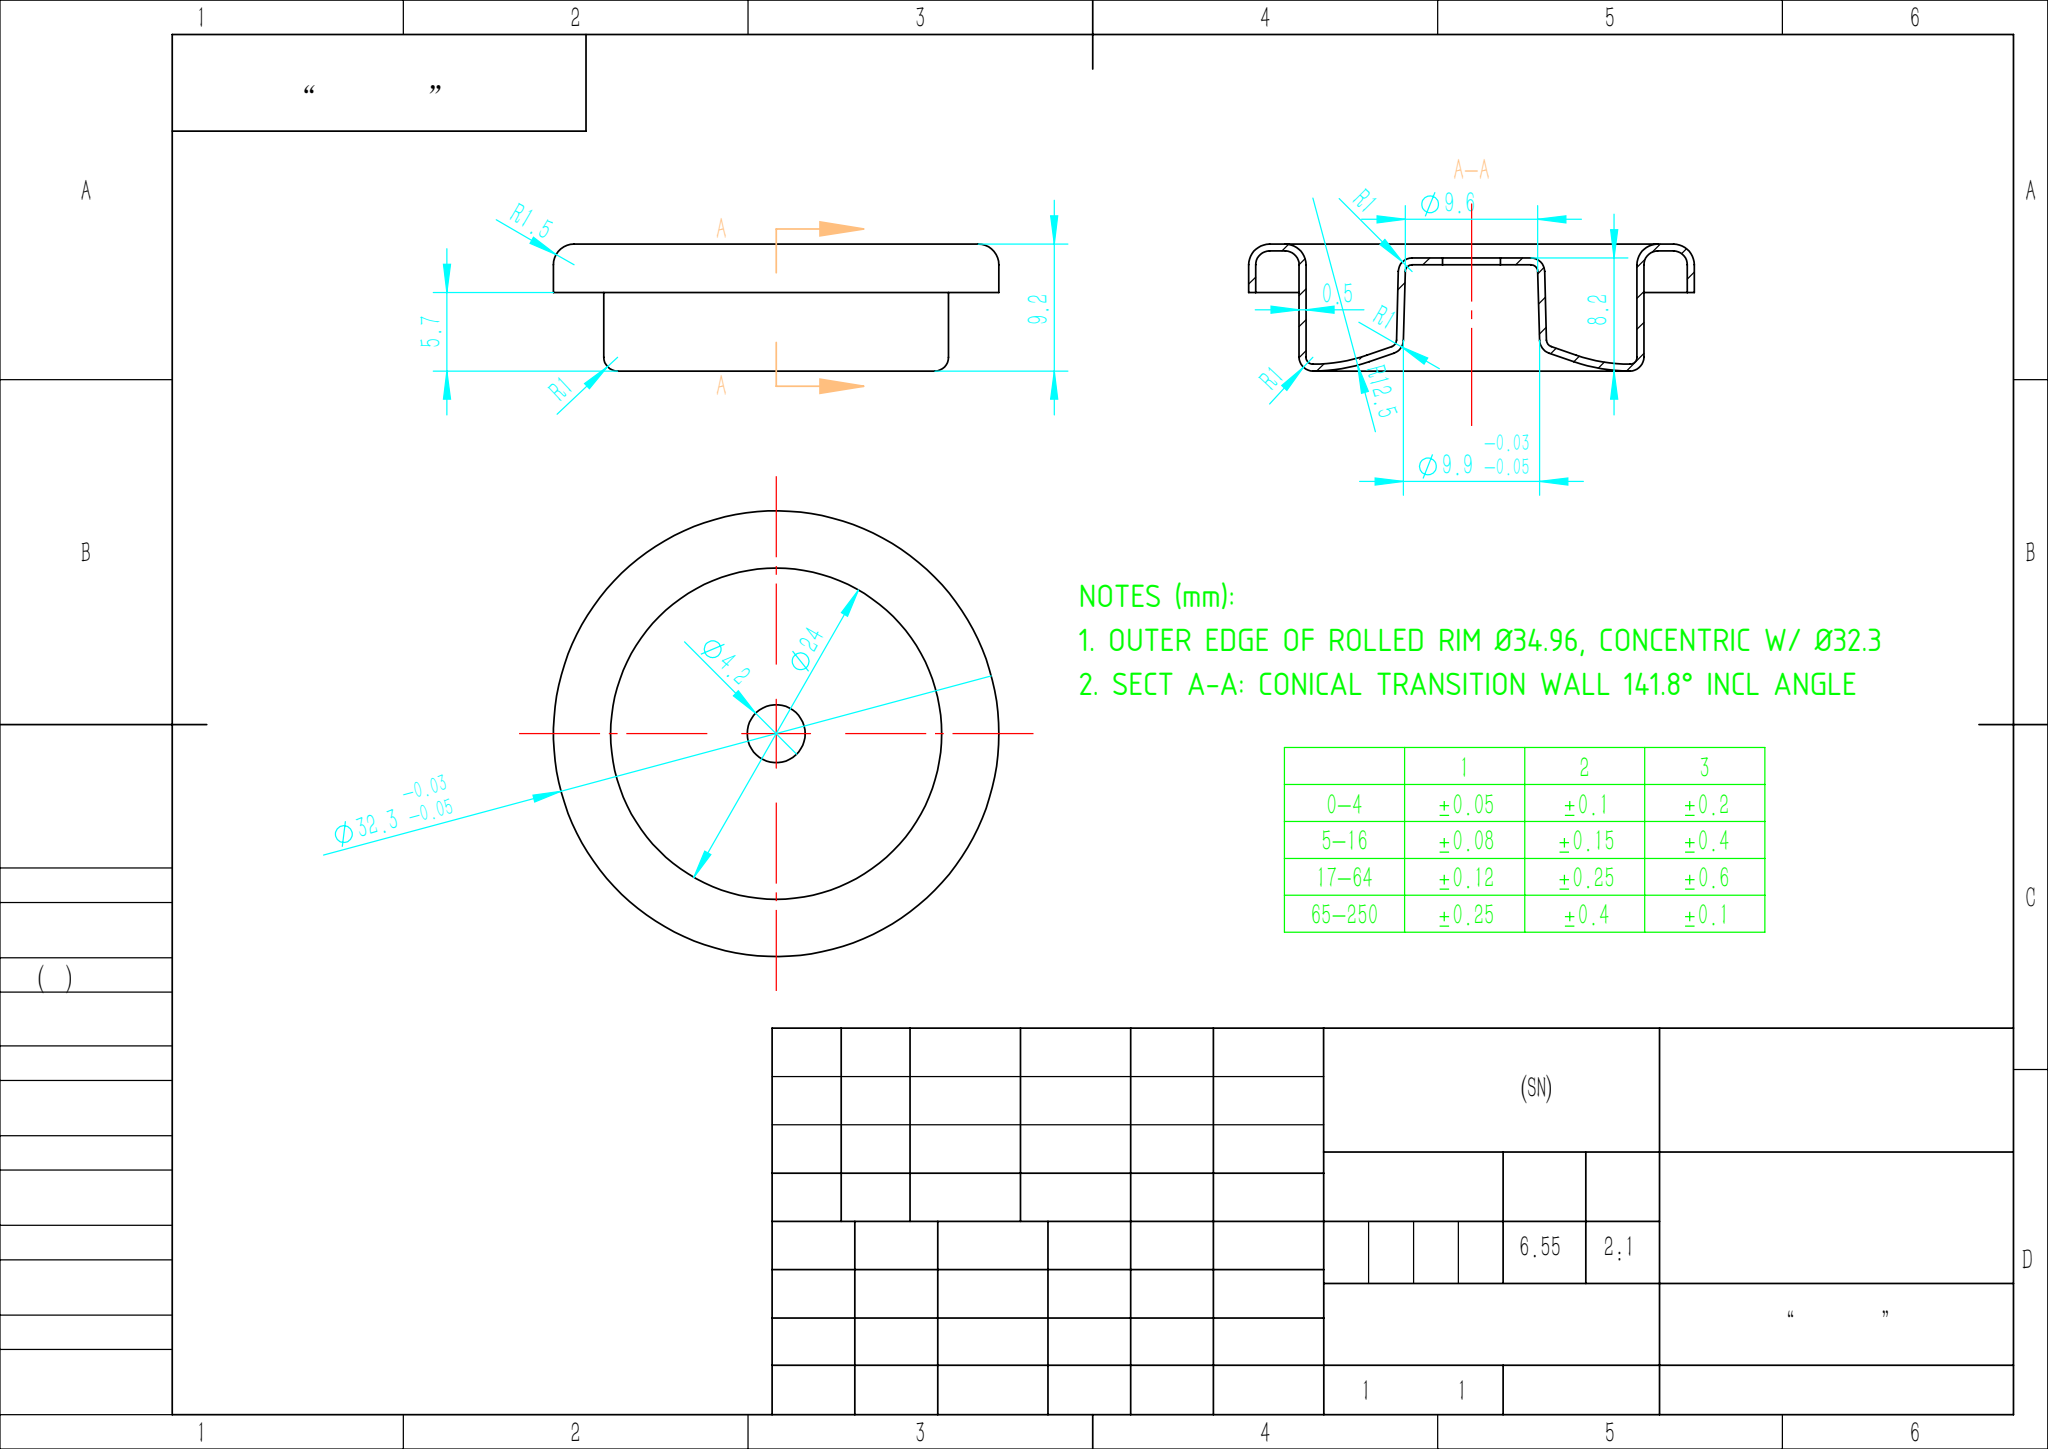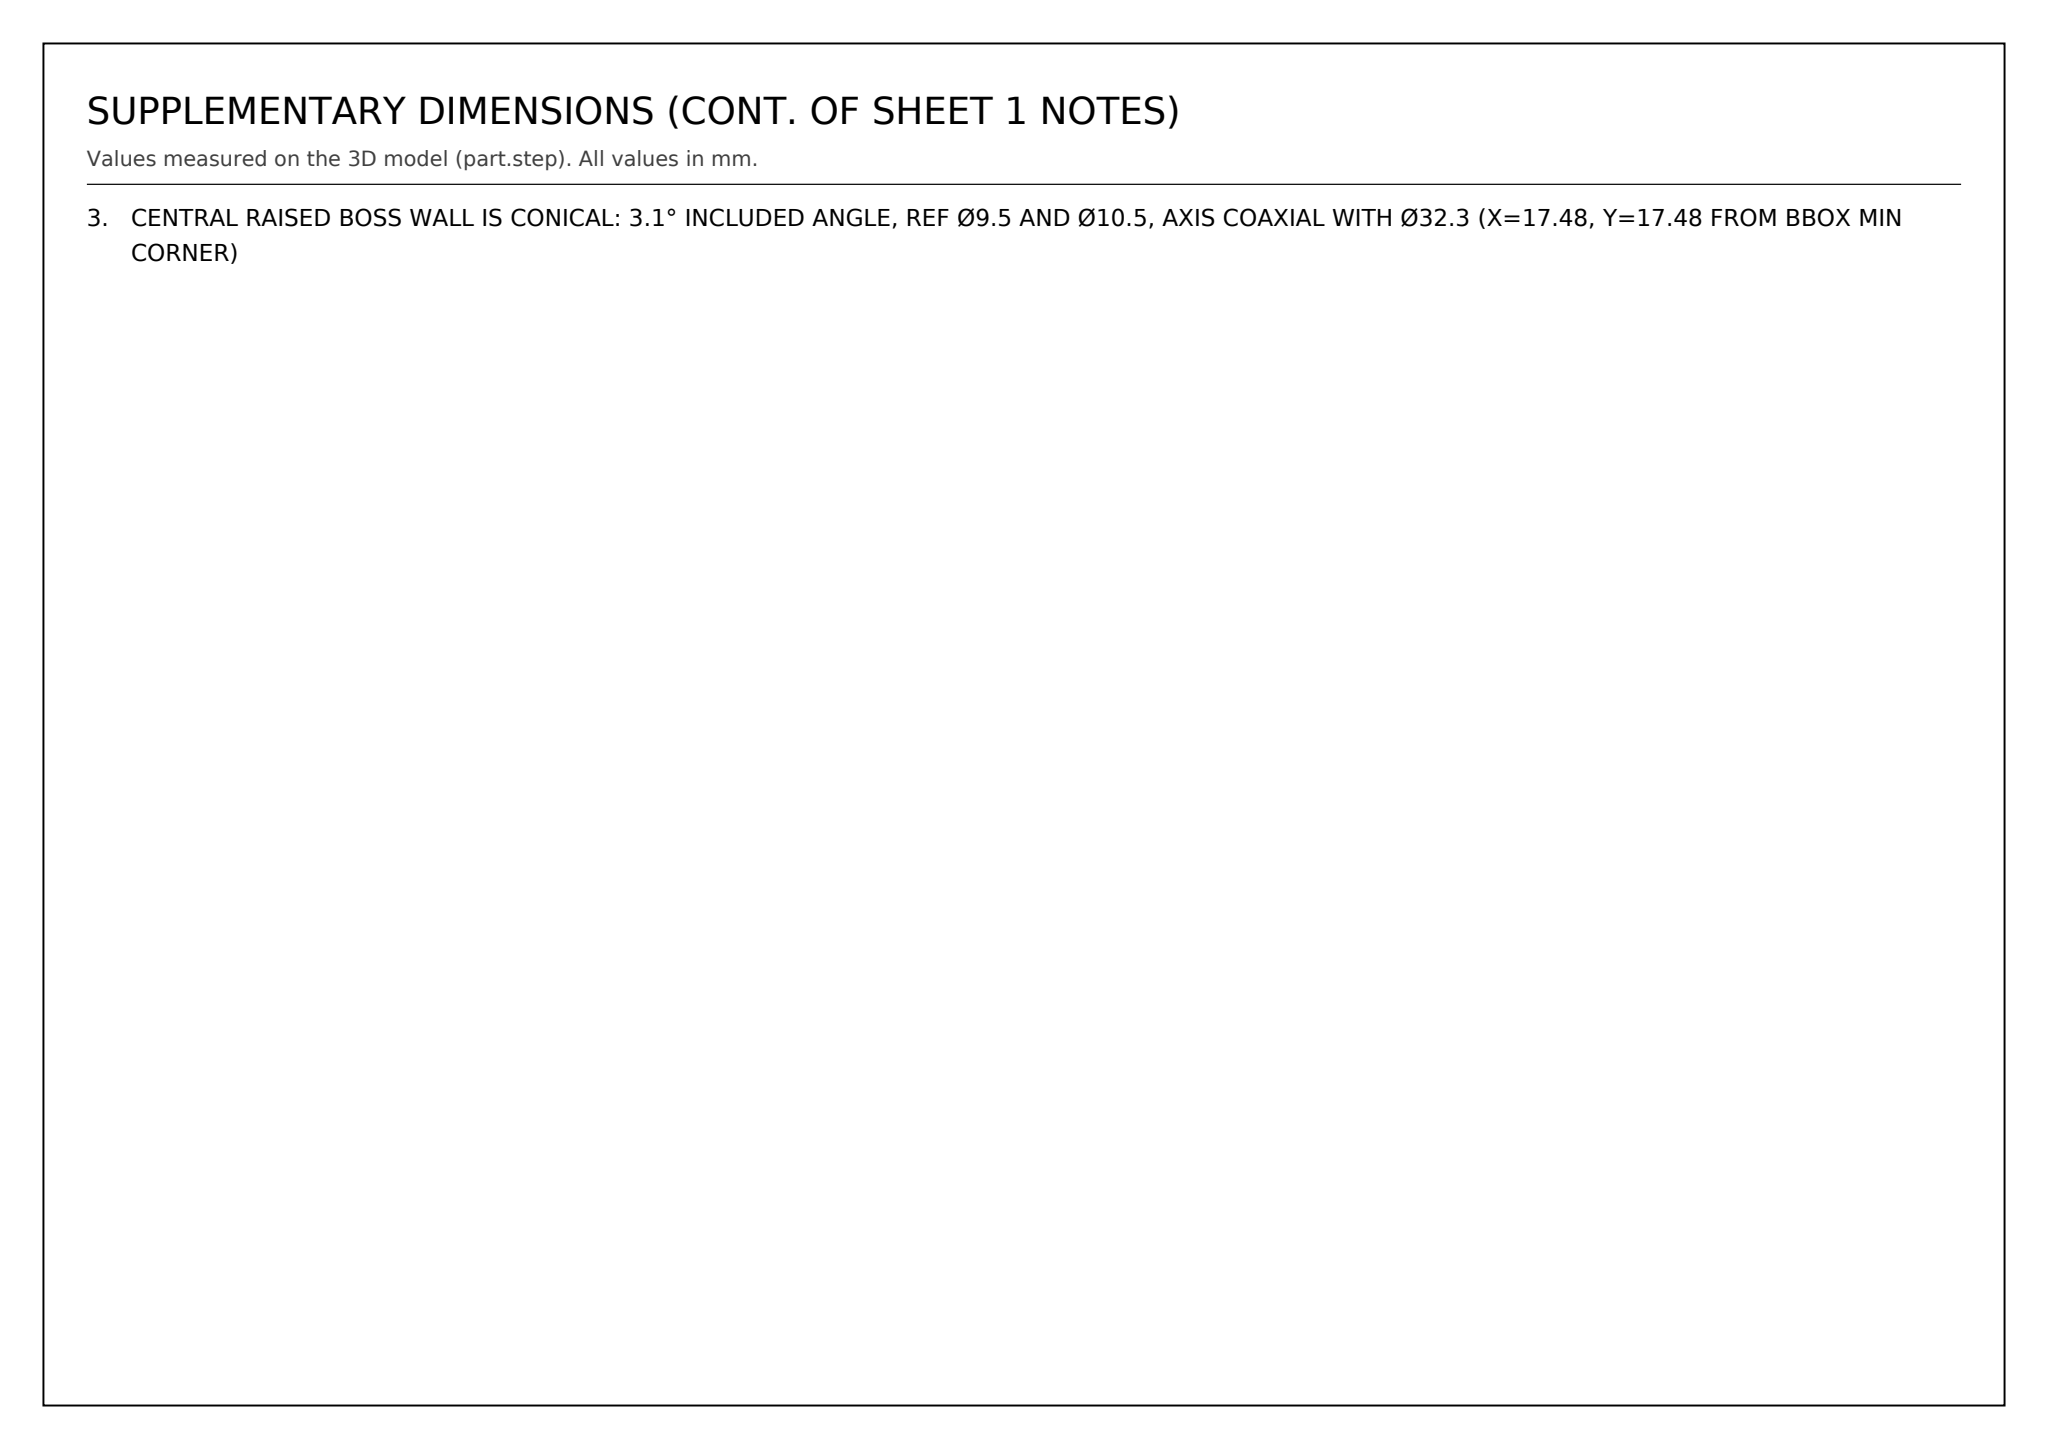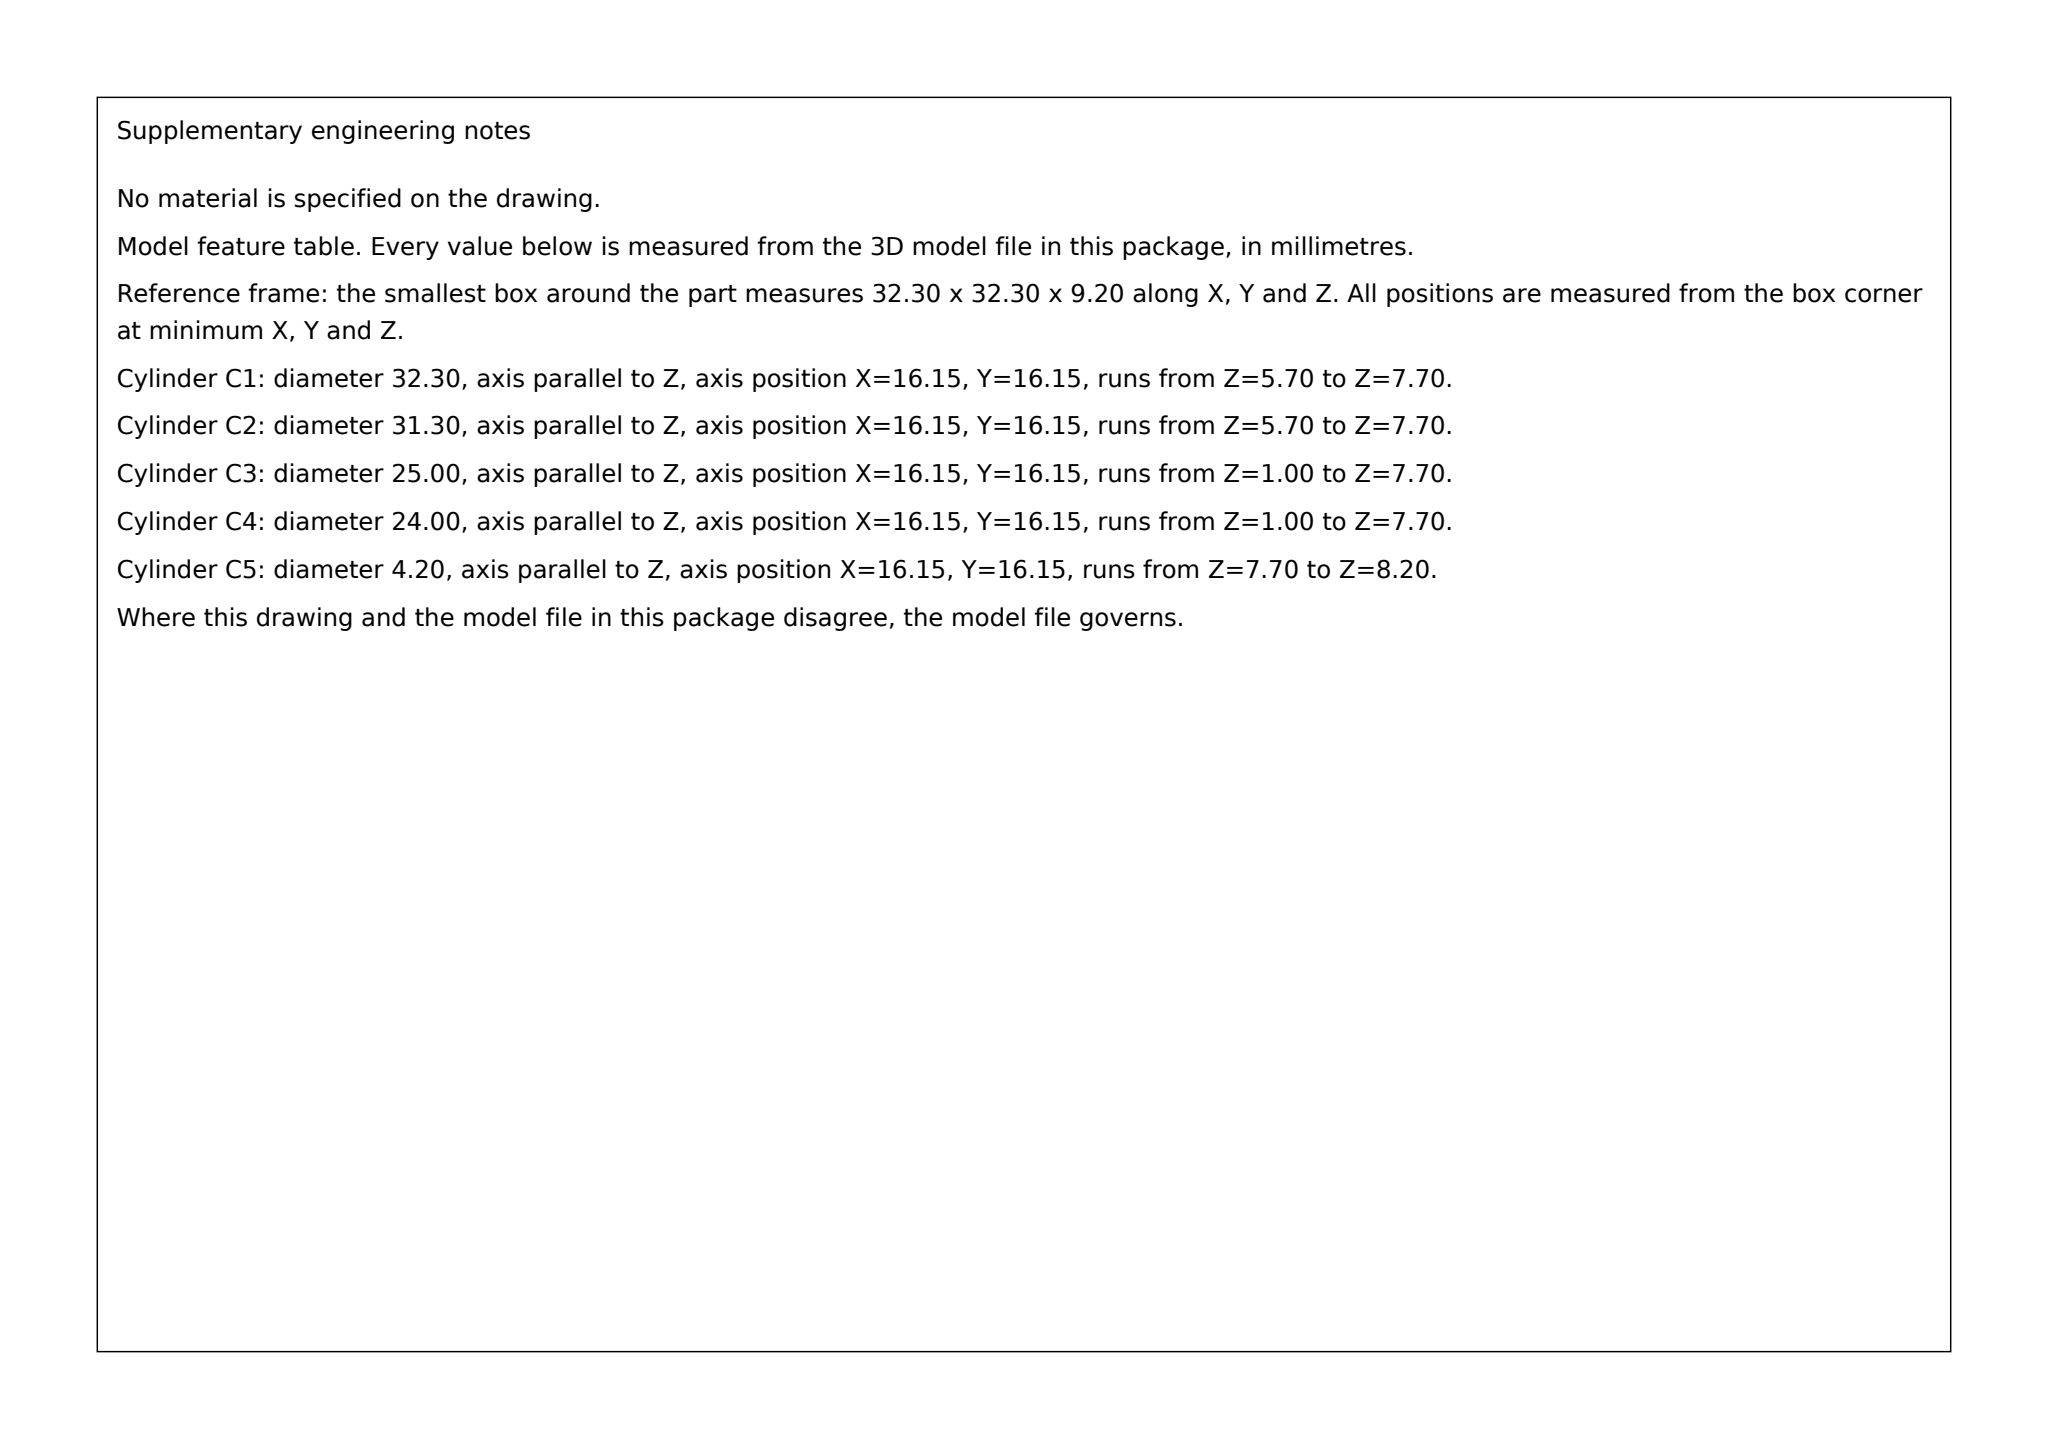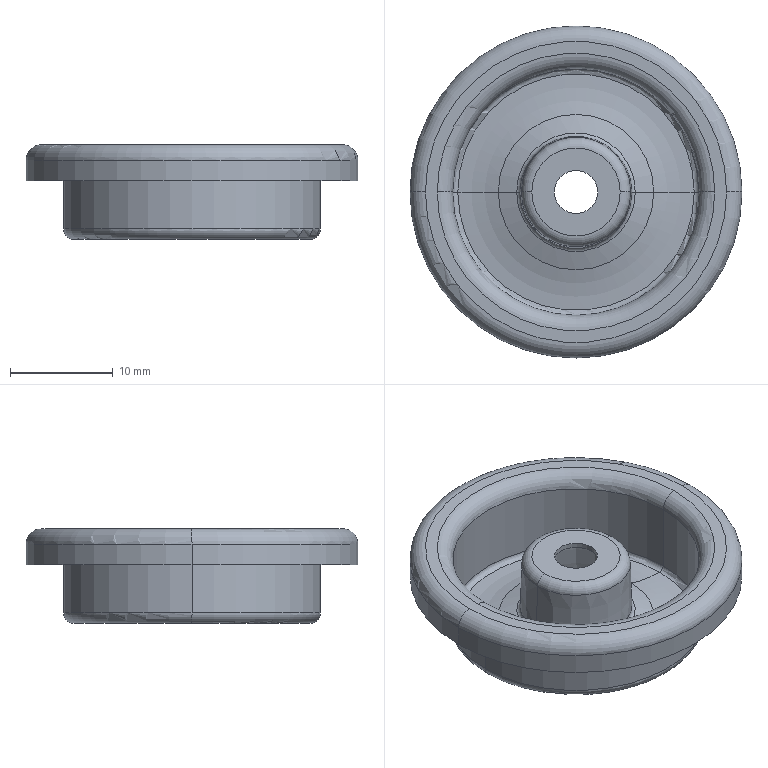Part | SolidWorks | mm | 1 solid | 47 faces | box 32.3 x 32.3 x 9.2 mm | volume 923 mm3 | torus 24 | cylinder 10 | cone 8 | plane 5 | commonest cylinder face diameters 4.2 x2 31.3 x2 32.3 x2 24 x2 25 x2
Drawing notes:
OUTER EDGE OF ROLLED RIM Ø34.96, CONCENTRIC W/ Ø32.3 | from the solid: bbox_xyz 34.961 x 34.961 about axis at (17.48,17.48); largest cyl called out is Ø32.3
SECT A-A: CONICAL TRANSITION WALL 141.8° INCL ANGLE | from the solid: cones[included_angle,ref_dia]: [141.8, 8.752] and [141.8, 8.425], 2 ea
CENTRAL RAISED BOSS WALL IS CONICAL: 3.1° INCLUDED ANGLE, REF Ø9.5 AND Ø10.5, AXIS COAXIAL WITH Ø32.3 (X=17.48, Y=17.48 FROM BBOX MIN CORNER) | from the solid: cones[included_angle,ref_dia]: [3.1, 10.5, 2] and [3.1, 9.5, 2]; cylinders Ø32.3 axis z at pos (17.48, 17.48)